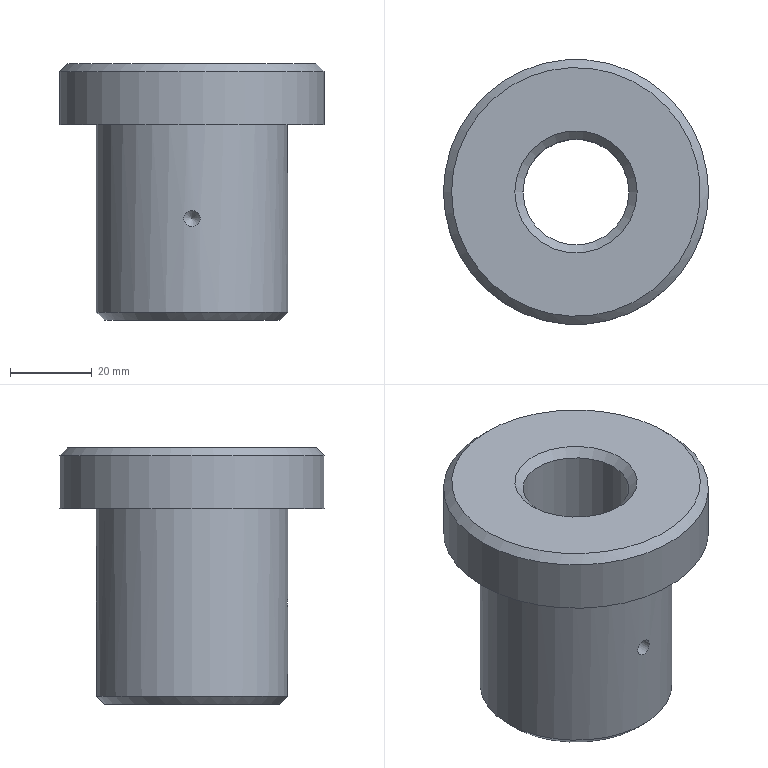Component | NX | BEARINGNUT | 1 solid | 12 faces | box 65 x 65 x 63 mm | volume 98521 mm3 | cone 5 | cylinder 4 | plane 3 | commonest cylinder face diameters 47 x1 65 x1 26 x1 4 x1
STEP:
#1=CARTESIAN_POINT('',(0.,0.,0.));
#2=DIRECTION('',(0.,0.,1.));
#3=DIRECTION('',(1.,0.,0.));
#4=AXIS2_PLACEMENT_3D('',#1,#2,#3);
#5=CARTESIAN_POINT('',(19.835,7.63,211.));
#6=VERTEX_POINT('',#5);
#7=CARTESIAN_POINT('',(4.835,7.63,211.));
#8=DIRECTION('',(0.,0.,1.));
#9=DIRECTION('',(1.,0.,0.));
#10=AXIS2_PLACEMENT_3D('',#7,#8,#9);
#11=CIRCLE('',#10,15.);
#12=CARTESIAN_POINT('',(4.835,7.63,211.));
#13=DIRECTION('',(0.,0.,-1.));
#14=DIRECTION('',(1.,0.,0.));
#15=AXIS2_PLACEMENT_3D('',#12,#13,#14);
#16=PLANE('',#15);
#17=CARTESIAN_POINT('',(15.,-0.));
#18=CARTESIAN_POINT('',(15.,-25.981));
#19=CARTESIAN_POINT('',(-7.5,-12.99));
#20=CARTESIAN_POINT('',(-30.,-0.));
#21=CARTESIAN_POINT('',(-7.5,12.99));
#22=CARTESIAN_POINT('',(15.,25.981));
#23=CARTESIAN_POINT('',(15.,-0.));
#24=(BOUNDED_CURVE()B_SPLINE_CURVE(2,(#17,#18,#19,#20,#21,#22,#23),.UNSPECIFIED.,.T.,.F.)B_SPLINE_CURVE_WITH_KNOTS((1,2,2,2,2,1),(-2.094,0.,2.094,4.189,6.283,8.378),.UNSPECIFIED.)CURVE()GEOMETRIC_REPRESENTATION_ITEM()RATIONAL_B_SPLINE_CURVE((1.,0.5,1.,0.5,1.,0.5,1.))REPRESENTATION_ITEM(''));
#25=(GEOMETRIC_REPRESENTATION_CONTEXT(2)PARAMETRIC_REPRESENTATION_CONTEXT()REPRESENTATION_CONTEXT('',''));
#26=DEFINITIONAL_REPRESENTATION('',(#24),#25);
#27=PCURVE('',#16,#26);
#28=CARTESIAN_POINT('',(4.835,7.63,213.));
#29=DIRECTION('',(0.,0.,-1.));
#30=DIRECTION('',(1.,0.,0.));
#31=AXIS2_PLACEMENT_3D('',#28,#29,#30);
#32=CONICAL_SURFACE('',#31,13.,0.7854);
#33=CARTESIAN_POINT('',(6.283,2.));
#34=DIRECTION('',(-1.,0.));
#35=VECTOR('',#34,1.);
#36=LINE('',#33,#35);
#37=(GEOMETRIC_REPRESENTATION_CONTEXT(2)PARAMETRIC_REPRESENTATION_CONTEXT()REPRESENTATION_CONTEXT('',''));
#38=DEFINITIONAL_REPRESENTATION('',(#36),#37);
#39=PCURVE('',#32,#38);
#40=SURFACE_CURVE('',#11,(#27,#39),.PCURVE_S1.);
#41=EDGE_CURVE('',#6,#6,#40,.T.);
#42=ORIENTED_EDGE('',*,*,#41,.T.);
#43=EDGE_LOOP('',(#42));
#44=FACE_BOUND('',#43,.T.);
#45=CARTESIAN_POINT('',(26.335,7.63,211.));
#46=VERTEX_POINT('',#45);
#47=CARTESIAN_POINT('',(4.835,7.63,211.));
#48=DIRECTION('',(0.,0.,-1.));
#49=DIRECTION('',(1.,0.,0.));
#50=AXIS2_PLACEMENT_3D('',#47,#48,#49);
#51=CIRCLE('',#50,21.5);
#52=CARTESIAN_POINT('',(0.,0.));
#53=DIRECTION('',(1.,0.));
#54=AXIS2_PLACEMENT_2D('',#52,#53);
#55=CIRCLE('',#54,21.5);
#56=(GEOMETRIC_REPRESENTATION_CONTEXT(2)PARAMETRIC_REPRESENTATION_CONTEXT()REPRESENTATION_CONTEXT('',''));
#57=DEFINITIONAL_REPRESENTATION('',(#55),#56);
#58=PCURVE('',#16,#57);
#59=CARTESIAN_POINT('',(4.835,7.63,213.));
#60=DIRECTION('',(0.,0.,1.));
#61=DIRECTION('',(-1.,0.,0.));
#62=AXIS2_PLACEMENT_3D('',#59,#60,#61);
#63=CONICAL_SURFACE('',#62,23.5,0.7854);
#64=CARTESIAN_POINT('',(9.425,-2.));
#65=DIRECTION('',(-1.,0.));
#66=VECTOR('',#65,1.);
#67=LINE('',#64,#66);
#68=(GEOMETRIC_REPRESENTATION_CONTEXT(2)PARAMETRIC_REPRESENTATION_CONTEXT()REPRESENTATION_CONTEXT('',''));
#69=DEFINITIONAL_REPRESENTATION('',(#67),#68);
#70=PCURVE('',#63,#69);
#71=SURFACE_CURVE('',#51,(#58,#70),.PCURVE_S1.);
#72=EDGE_CURVE('',#46,#46,#71,.T.);
#73=ORIENTED_EDGE('',*,*,#72,.T.);
#74=EDGE_LOOP('',(#73));
#75=FACE_BOUND('',#74,.T.);
#76=ADVANCED_FACE('',(#44,#75),#16,.T.);
#77=CARTESIAN_POINT('',(28.335,7.63,213.));
#78=VERTEX_POINT('',#77);
#79=CARTESIAN_POINT('',(-18.665,7.63,213.));
#80=VERTEX_POINT('',#79);
#81=CARTESIAN_POINT('',(4.835,7.63,213.));
#82=DIRECTION('',(0.,0.,1.));
#83=DIRECTION('',(1.,0.,0.));
#84=AXIS2_PLACEMENT_3D('',#81,#82,#83);
#85=CIRCLE('',#84,23.5);
#86=CARTESIAN_POINT('',(4.835,7.63,211.));
#87=DIRECTION('',(0.,0.,1.));
#88=DIRECTION('',(-1.,0.,0.));
#89=AXIS2_PLACEMENT_3D('',#86,#87,#88);
#90=CYLINDRICAL_SURFACE('',#89,23.5);
#91=CARTESIAN_POINT('',(3.142,2.));
#92=DIRECTION('',(1.,0.));
#93=VECTOR('',#92,1.);
#94=LINE('',#91,#93);
#95=(GEOMETRIC_REPRESENTATION_CONTEXT(2)PARAMETRIC_REPRESENTATION_CONTEXT()REPRESENTATION_CONTEXT('',''));
#96=DEFINITIONAL_REPRESENTATION('',(#94),#95);
#97=PCURVE('',#90,#96);
#98=CARTESIAN_POINT('',(3.142,0.));
#99=DIRECTION('',(1.,0.));
#100=VECTOR('',#99,1.);
#101=LINE('',#98,#100);
#102=(GEOMETRIC_REPRESENTATION_CONTEXT(2)PARAMETRIC_REPRESENTATION_CONTEXT()REPRESENTATION_CONTEXT('',''));
#103=DEFINITIONAL_REPRESENTATION('',(#101),#102);
#104=PCURVE('',#63,#103);
#105=SURFACE_CURVE('',#85,(#97,#104),.PCURVE_S1.);
#106=EDGE_CURVE('',#78,#80,#105,.T.);
#107=ORIENTED_EDGE('',*,*,#106,.T.);
#108=CARTESIAN_POINT('',(-18.665,7.63,259.));
#109=VERTEX_POINT('',#108);
#110=CARTESIAN_POINT('',(-18.665,7.63,213.));
#111=CARTESIAN_POINT('',(-18.665,7.63,259.));
#112=B_SPLINE_CURVE_WITH_KNOTS('',1,(#110,#111),.UNSPECIFIED.,.F.,.F.,(2,2),(2.,48.),.PIECEWISE_BEZIER_KNOTS.);
#113=CARTESIAN_POINT('',(6.283,0.));
#114=DIRECTION('',(0.,1.));
#115=VECTOR('',#114,1.);
#116=LINE('',#113,#115);
#117=(GEOMETRIC_REPRESENTATION_CONTEXT(2)PARAMETRIC_REPRESENTATION_CONTEXT()REPRESENTATION_CONTEXT('',''));
#118=DEFINITIONAL_REPRESENTATION('',(#116),#117);
#119=PCURVE('',#90,#118);
#120=CARTESIAN_POINT('',(0.,0.));
#121=DIRECTION('',(0.,1.));
#122=VECTOR('',#121,1.);
#123=LINE('',#120,#122);
#124=(GEOMETRIC_REPRESENTATION_CONTEXT(2)PARAMETRIC_REPRESENTATION_CONTEXT()REPRESENTATION_CONTEXT('',''));
#125=DEFINITIONAL_REPRESENTATION('',(#123),#124);
#126=PCURVE('',#90,#125);
#127=SEAM_CURVE('',#112,(#119,#126),.PCURVE_S1.);
#128=EDGE_CURVE('',#80,#109,#127,.T.);
#129=ORIENTED_EDGE('',*,*,#128,.T.);
#130=CARTESIAN_POINT('',(4.835,7.63,259.));
#131=DIRECTION('',(0.,0.,-1.));
#132=DIRECTION('',(-1.,0.,0.));
#133=AXIS2_PLACEMENT_3D('',#130,#131,#132);
#134=CIRCLE('',#133,23.5);
#135=CARTESIAN_POINT('',(6.283,48.));
#136=DIRECTION('',(-1.,0.));
#137=VECTOR('',#136,1.);
#138=LINE('',#135,#137);
#139=(GEOMETRIC_REPRESENTATION_CONTEXT(2)PARAMETRIC_REPRESENTATION_CONTEXT()REPRESENTATION_CONTEXT('',''));
#140=DEFINITIONAL_REPRESENTATION('',(#138),#139);
#141=PCURVE('',#90,#140);
#142=CARTESIAN_POINT('',(4.835,7.63,259.));
#143=DIRECTION('',(0.,0.,-1.));
#144=DIRECTION('',(1.,0.,0.));
#145=AXIS2_PLACEMENT_3D('',#142,#143,#144);
#146=PLANE('',#145);
#147=CARTESIAN_POINT('',(0.,0.));
#148=DIRECTION('',(-1.,0.));
#149=AXIS2_PLACEMENT_2D('',#147,#148);
#150=CIRCLE('',#149,23.5);
#151=(GEOMETRIC_REPRESENTATION_CONTEXT(2)PARAMETRIC_REPRESENTATION_CONTEXT()REPRESENTATION_CONTEXT('',''));
#152=DEFINITIONAL_REPRESENTATION('',(#150),#151);
#153=PCURVE('',#146,#152);
#154=SURFACE_CURVE('',#134,(#141,#153),.PCURVE_S1.);
#155=EDGE_CURVE('',#109,#109,#154,.T.);
#156=ORIENTED_EDGE('',*,*,#155,.T.);
#157=ORIENTED_EDGE('',*,*,#128,.F.);
#158=CARTESIAN_POINT('',(4.835,7.63,213.));
#159=DIRECTION('',(0.,0.,1.));
#160=DIRECTION('',(1.,0.,0.));
#161=AXIS2_PLACEMENT_3D('',#158,#159,#160);
#162=CIRCLE('',#161,23.5);
#163=CARTESIAN_POINT('',(-3.142,2.));
#164=DIRECTION('',(1.,0.));
#165=VECTOR('',#164,1.);
#166=LINE('',#163,#165);
#167=(GEOMETRIC_REPRESENTATION_CONTEXT(2)PARAMETRIC_REPRESENTATION_CONTEXT()REPRESENTATION_CONTEXT('',''));
#168=DEFINITIONAL_REPRESENTATION('',(#166),#167);
#169=PCURVE('',#90,#168);
#170=CARTESIAN_POINT('',(3.142,0.));
#171=DIRECTION('',(1.,0.));
#172=VECTOR('',#171,1.);
#173=LINE('',#170,#172);
#174=(GEOMETRIC_REPRESENTATION_CONTEXT(2)PARAMETRIC_REPRESENTATION_CONTEXT()REPRESENTATION_CONTEXT('',''));
#175=DEFINITIONAL_REPRESENTATION('',(#173),#174);
#176=PCURVE('',#63,#175);
#177=SURFACE_CURVE('',#162,(#169,#176),.PCURVE_S1.);
#178=EDGE_CURVE('',#80,#78,#177,.T.);
#179=ORIENTED_EDGE('',*,*,#178,.T.);
#180=EDGE_LOOP('',(#107,#129,#156,#157,#179));
#181=FACE_BOUND('',#180,.T.);
#182=CARTESIAN_POINT('',(4.835,-15.87,234.));
#183=VERTEX_POINT('',#182);
#184=CARTESIAN_POINT('',(4.835,-15.87,234.));
#185=CARTESIAN_POINT('',(5.059,-15.87,234.));
#186=CARTESIAN_POINT('',(5.285,-15.866,234.038));
#187=CARTESIAN_POINT('',(5.496,-15.86,234.112));
#188=CARTESIAN_POINT('',(5.707,-15.854,234.186));
#189=CARTESIAN_POINT('',(5.908,-15.846,234.297));
#190=CARTESIAN_POINT('',(6.082,-15.837,234.436));
#191=CARTESIAN_POINT('',(6.257,-15.827,234.576));
#192=CARTESIAN_POINT('',(6.41,-15.817,234.747));
#193=CARTESIAN_POINT('',(6.529,-15.808,234.937));
#194=CARTESIAN_POINT('',(6.648,-15.8,235.126));
#195=CARTESIAN_POINT('',(6.736,-15.793,235.339));
#196=CARTESIAN_POINT('',(6.786,-15.789,235.558));
#197=CARTESIAN_POINT('',(6.835,-15.784,235.776));
#198=CARTESIAN_POINT('',(6.848,-15.783,236.006));
#199=CARTESIAN_POINT('',(6.822,-15.785,236.228));
#200=CARTESIAN_POINT('',(6.797,-15.788,236.45));
#201=CARTESIAN_POINT('',(6.733,-15.793,236.67));
#202=CARTESIAN_POINT('',(6.636,-15.801,236.871));
#203=CARTESIAN_POINT('',(6.539,-15.808,237.072));
#204=CARTESIAN_POINT('',(6.405,-15.818,237.259));
#205=CARTESIAN_POINT('',(6.247,-15.827,237.416));
#206=CARTESIAN_POINT('',(6.089,-15.837,237.574));
#207=CARTESIAN_POINT('',(5.901,-15.846,237.707));
#208=CARTESIAN_POINT('',(5.699,-15.854,237.804));
#209=CARTESIAN_POINT('',(5.497,-15.861,237.901));
#210=CARTESIAN_POINT('',(5.275,-15.867,237.964));
#211=CARTESIAN_POINT('',(5.052,-15.869,237.988));
#212=CARTESIAN_POINT('',(4.83,-15.871,238.012));
#213=CARTESIAN_POINT('',(4.601,-15.869,237.999));
#214=CARTESIAN_POINT('',(4.383,-15.865,237.948));
#215=CARTESIAN_POINT('',(4.166,-15.861,237.898));
#216=CARTESIAN_POINT('',(3.955,-15.854,237.809));
#217=CARTESIAN_POINT('',(3.766,-15.845,237.69));
#218=CARTESIAN_POINT('',(3.577,-15.837,237.571));
#219=CARTESIAN_POINT('',(3.406,-15.827,237.417));
#220=CARTESIAN_POINT('',(3.268,-15.817,237.242));
#221=CARTESIAN_POINT('',(3.129,-15.808,237.067));
#222=CARTESIAN_POINT('',(3.018,-15.799,236.864));
#223=CARTESIAN_POINT('',(2.945,-15.793,236.653));
#224=CARTESIAN_POINT('',(2.872,-15.788,236.441));
#225=CARTESIAN_POINT('',(2.834,-15.784,236.214));
#226=CARTESIAN_POINT('',(2.835,-15.784,235.99));
#227=CARTESIAN_POINT('',(2.836,-15.784,235.767));
#228=CARTESIAN_POINT('',(2.876,-15.788,235.541));
#229=CARTESIAN_POINT('',(2.951,-15.794,235.33));
#230=CARTESIAN_POINT('',(3.025,-15.8,235.12));
#231=CARTESIAN_POINT('',(3.137,-15.809,234.92));
#232=CARTESIAN_POINT('',(3.277,-15.818,234.746));
#233=CARTESIAN_POINT('',(3.417,-15.827,234.572));
#234=CARTESIAN_POINT('',(3.589,-15.837,234.419));
#235=CARTESIAN_POINT('',(3.779,-15.846,234.301));
#236=CARTESIAN_POINT('',(3.97,-15.854,234.183));
#237=CARTESIAN_POINT('',(4.183,-15.862,234.096));
#238=CARTESIAN_POINT('',(4.402,-15.866,234.047));
#239=CARTESIAN_POINT('',(4.544,-15.868,234.016));
#240=CARTESIAN_POINT('',(4.69,-15.87,234.));
#241=CARTESIAN_POINT('',(4.835,-15.87,234.));
#242=B_SPLINE_CURVE_WITH_KNOTS('',3,(#184,#185,#186,#187,#188,#189,#190,#191,#192,#193,#194,#195,#196,#197,#198,#199,#200,#201,#202,#203,#204,#205,#206,#207,#208,#209,#210,#211,#212,#213,#214,#215,#216,#217,#218,#219,#220,#221,#222,#223,#224,#225,#226,#227,#228,#229,#230,#231,#232,#233,#234,#235,#236,#237,#238,#239,#240,#241),.UNSPECIFIED.,.T.,.F.,(1,3,3,3,3,3,3,3,3,3,3,3,3,3,3,3,3,3,3,3,3,1),(-0.03454,0.,0.05357,0.1071,0.1608,0.2146,0.2682,0.3217,0.3753,0.429,0.4828,0.5364,0.5899,0.6435,0.6973,0.751,0.8045,0.858,0.9117,0.9655,1.,1.054),.UNSPECIFIED.);
#243=CARTESIAN_POINT('',(1.571,23.));
#244=CARTESIAN_POINT('',(1.573,23.));
#245=CARTESIAN_POINT('',(1.577,23.003));
#246=CARTESIAN_POINT('',(1.583,23.019));
#247=CARTESIAN_POINT('',(1.589,23.044));
#248=CARTESIAN_POINT('',(1.595,23.08));
#249=CARTESIAN_POINT('',(1.601,23.124));
#250=CARTESIAN_POINT('',(1.606,23.179));
#251=CARTESIAN_POINT('',(1.612,23.243));
#252=CARTESIAN_POINT('',(1.617,23.316));
#253=CARTESIAN_POINT('',(1.622,23.398));
#254=CARTESIAN_POINT('',(1.627,23.487));
#255=CARTESIAN_POINT('',(1.631,23.584));
#256=CARTESIAN_POINT('',(1.635,23.689));
#257=CARTESIAN_POINT('',(1.639,23.8));
#258=CARTESIAN_POINT('',(1.643,23.917));
#259=CARTESIAN_POINT('',(1.646,24.04));
#260=CARTESIAN_POINT('',(1.648,24.168));
#261=CARTESIAN_POINT('',(1.651,24.3));
#262=CARTESIAN_POINT('',(1.653,24.436));
#263=CARTESIAN_POINT('',(1.654,24.574));
#264=CARTESIAN_POINT('',(1.655,24.714));
#265=CARTESIAN_POINT('',(1.656,24.856));
#266=CARTESIAN_POINT('',(1.656,25.));
#267=CARTESIAN_POINT('',(1.656,25.143));
#268=CARTESIAN_POINT('',(1.655,25.284));
#269=CARTESIAN_POINT('',(1.654,25.425));
#270=CARTESIAN_POINT('',(1.653,25.563));
#271=CARTESIAN_POINT('',(1.651,25.699));
#272=CARTESIAN_POINT('',(1.648,25.831));
#273=CARTESIAN_POINT('',(1.646,25.958));
#274=CARTESIAN_POINT('',(1.643,26.081));
#275=CARTESIAN_POINT('',(1.639,26.199));
#276=CARTESIAN_POINT('',(1.635,26.31));
#277=CARTESIAN_POINT('',(1.631,26.415));
#278=CARTESIAN_POINT('',(1.627,26.512));
#279=CARTESIAN_POINT('',(1.622,26.602));
#280=CARTESIAN_POINT('',(1.617,26.683));
#281=CARTESIAN_POINT('',(1.612,26.756));
#282=CARTESIAN_POINT('',(1.606,26.82));
#283=CARTESIAN_POINT('',(1.601,26.875));
#284=CARTESIAN_POINT('',(1.595,26.92));
#285=CARTESIAN_POINT('',(1.589,26.956));
#286=CARTESIAN_POINT('',(1.583,26.981));
#287=CARTESIAN_POINT('',(1.577,26.996));
#288=CARTESIAN_POINT('',(1.571,27.002));
#289=CARTESIAN_POINT('',(1.565,26.996));
#290=CARTESIAN_POINT('',(1.559,26.981));
#291=CARTESIAN_POINT('',(1.553,26.956));
#292=CARTESIAN_POINT('',(1.547,26.921));
#293=CARTESIAN_POINT('',(1.541,26.876));
#294=CARTESIAN_POINT('',(1.535,26.821));
#295=CARTESIAN_POINT('',(1.53,26.757));
#296=CARTESIAN_POINT('',(1.525,26.685));
#297=CARTESIAN_POINT('',(1.52,26.603));
#298=CARTESIAN_POINT('',(1.515,26.514));
#299=CARTESIAN_POINT('',(1.511,26.416));
#300=CARTESIAN_POINT('',(1.506,26.312));
#301=CARTESIAN_POINT('',(1.503,26.201));
#302=CARTESIAN_POINT('',(1.499,26.084));
#303=CARTESIAN_POINT('',(1.496,25.961));
#304=CARTESIAN_POINT('',(1.493,25.833));
#305=CARTESIAN_POINT('',(1.491,25.701));
#306=CARTESIAN_POINT('',(1.489,25.566));
#307=CARTESIAN_POINT('',(1.487,25.428));
#308=CARTESIAN_POINT('',(1.486,25.287));
#309=CARTESIAN_POINT('',(1.486,25.144));
#310=CARTESIAN_POINT('',(1.486,25.002));
#311=CARTESIAN_POINT('',(1.486,24.859));
#312=CARTESIAN_POINT('',(1.486,24.717));
#313=CARTESIAN_POINT('',(1.487,24.576));
#314=CARTESIAN_POINT('',(1.489,24.437));
#315=CARTESIAN_POINT('',(1.491,24.302));
#316=CARTESIAN_POINT('',(1.493,24.17));
#317=CARTESIAN_POINT('',(1.496,24.042));
#318=CARTESIAN_POINT('',(1.499,23.919));
#319=CARTESIAN_POINT('',(1.503,23.802));
#320=CARTESIAN_POINT('',(1.506,23.691));
#321=CARTESIAN_POINT('',(1.51,23.586));
#322=CARTESIAN_POINT('',(1.515,23.489));
#323=CARTESIAN_POINT('',(1.52,23.399));
#324=CARTESIAN_POINT('',(1.525,23.317));
#325=CARTESIAN_POINT('',(1.53,23.245));
#326=CARTESIAN_POINT('',(1.535,23.18));
#327=CARTESIAN_POINT('',(1.541,23.126));
#328=CARTESIAN_POINT('',(1.547,23.08));
#329=CARTESIAN_POINT('',(1.553,23.045));
#330=CARTESIAN_POINT('',(1.559,23.019));
#331=CARTESIAN_POINT('',(1.565,23.003));
#332=CARTESIAN_POINT('',(1.569,23.));
#333=CARTESIAN_POINT('',(1.571,23.));
#334=B_SPLINE_CURVE_WITH_KNOTS('',3,(#243,#244,#245,#246,#247,#248,#249,#250,#251,#252,#253,#254,#255,#256,#257,#258,#259,#260,#261,#262,#263,#264,#265,#266,#267,#268,#269,#270,#271,#272,#273,#274,#275,#276,#277,#278,#279,#280,#281,#282,#283,#284,#285,#286,#287,#288,#289,#290,#291,#292,#293,#294,#295,#296,#297,#298,#299,#300,#301,#302,#303,#304,#305,#306,#307,#308,#309,#310,#311,#312,#313,#314,#315,#316,#317,#318,#319,#320,#321,#322,#323,#324,#325,#326,#327,#328,#329,#330,#331,#332,#333),.UNSPECIFIED.,.T.,.F.,(4,1,1,1,1,1,1,1,1,1,1,1,1,1,1,1,1,1,1,1,1,1,1,1,1,1,1,1,1,1,1,1,1,1,1,1,1,1,1,1,1,1,1,1,1,1,1,1,1,1,1,1,1,1,1,1,1,1,1,1,1,1,1,1,1,1,1,1,1,1,1,1,1,1,1,1,1,1,1,1,1,1,1,1,1,1,1,1,4),(0.,0.01136,0.02273,0.03409,0.04545,0.05682,0.06818,0.07955,0.09091,0.1023,0.1136,0.125,0.1364,0.1477,0.1591,0.1705,0.1818,0.1932,0.2045,0.2159,0.2273,0.2386,0.25,0.2614,0.2727,0.2841,0.2955,0.3068,0.3182,0.3295,0.3409,0.3523,0.3636,0.375,0.3864,0.3977,0.4091,0.4205,0.4318,0.4432,0.4545,0.4659,0.4773,0.4886,0.5,0.5114,0.5227,0.5341,0.5455,0.5568,0.5682,0.5795,0.5909,0.6023,0.6136,0.625,0.6364,0.6477,0.6591,0.6705,0.6818,0.6932,0.7045,0.7159,0.7273,0.7386,0.75,0.7614,0.7727,0.7841,0.7955,0.8068,0.8182,0.8295,0.8409,0.8523,0.8636,0.875,0.8864,0.8977,0.9091,0.9205,0.9318,0.9432,0.9545,0.9659,0.9773,0.9886,1.),.QUASI_UNIFORM_KNOTS.);
#335=(GEOMETRIC_REPRESENTATION_CONTEXT(2)PARAMETRIC_REPRESENTATION_CONTEXT()REPRESENTATION_CONTEXT('',''));
#336=DEFINITIONAL_REPRESENTATION('',(#334),#335);
#337=PCURVE('',#90,#336);
#338=CARTESIAN_POINT('',(4.835,-70.37,236.));
#339=DIRECTION('',(0.,1.,0.));
#340=DIRECTION('',(0.,0.,-1.));
#341=AXIS2_PLACEMENT_3D('',#338,#339,#340);
#342=CYLINDRICAL_SURFACE('',#341,2.);
#343=CARTESIAN_POINT('',(6.283,54.5));
#344=CARTESIAN_POINT('',(6.259,54.5));
#345=CARTESIAN_POINT('',(6.212,54.5));
#346=CARTESIAN_POINT('',(6.14,54.502));
#347=CARTESIAN_POINT('',(6.069,54.504));
#348=CARTESIAN_POINT('',(5.997,54.507));
#349=CARTESIAN_POINT('',(5.926,54.51));
#350=CARTESIAN_POINT('',(5.855,54.515));
#351=CARTESIAN_POINT('',(5.783,54.519));
#352=CARTESIAN_POINT('',(5.712,54.525));
#353=CARTESIAN_POINT('',(5.64,54.531));
#354=CARTESIAN_POINT('',(5.569,54.536));
#355=CARTESIAN_POINT('',(5.498,54.543));
#356=CARTESIAN_POINT('',(5.427,54.549));
#357=CARTESIAN_POINT('',(5.355,54.555));
#358=CARTESIAN_POINT('',(5.284,54.56));
#359=CARTESIAN_POINT('',(5.213,54.566));
#360=CARTESIAN_POINT('',(5.141,54.571));
#361=CARTESIAN_POINT('',(5.07,54.575));
#362=CARTESIAN_POINT('',(4.998,54.579));
#363=CARTESIAN_POINT('',(4.927,54.582));
#364=CARTESIAN_POINT('',(4.856,54.584));
#365=CARTESIAN_POINT('',(4.784,54.585));
#366=CARTESIAN_POINT('',(4.713,54.585));
#367=CARTESIAN_POINT('',(4.641,54.585));
#368=CARTESIAN_POINT('',(4.57,54.584));
#369=CARTESIAN_POINT('',(4.499,54.582));
#370=CARTESIAN_POINT('',(4.427,54.579));
#371=CARTESIAN_POINT('',(4.355,54.575));
#372=CARTESIAN_POINT('',(4.284,54.571));
#373=CARTESIAN_POINT('',(4.213,54.566));
#374=CARTESIAN_POINT('',(4.142,54.56));
#375=CARTESIAN_POINT('',(4.07,54.555));
#376=CARTESIAN_POINT('',(3.999,54.549));
#377=CARTESIAN_POINT('',(3.927,54.543));
#378=CARTESIAN_POINT('',(3.856,54.537));
#379=CARTESIAN_POINT('',(3.785,54.531));
#380=CARTESIAN_POINT('',(3.713,54.525));
#381=CARTESIAN_POINT('',(3.642,54.52));
#382=CARTESIAN_POINT('',(3.571,54.515));
#383=CARTESIAN_POINT('',(3.499,54.51));
#384=CARTESIAN_POINT('',(3.428,54.507));
#385=CARTESIAN_POINT('',(3.356,54.504));
#386=CARTESIAN_POINT('',(3.285,54.502));
#387=CARTESIAN_POINT('',(3.214,54.5));
#388=CARTESIAN_POINT('',(3.142,54.5));
#389=CARTESIAN_POINT('',(3.071,54.5));
#390=CARTESIAN_POINT('',(2.999,54.502));
#391=CARTESIAN_POINT('',(2.928,54.504));
#392=CARTESIAN_POINT('',(2.857,54.507));
#393=CARTESIAN_POINT('',(2.785,54.51));
#394=CARTESIAN_POINT('',(2.714,54.515));
#395=CARTESIAN_POINT('',(2.642,54.519));
#396=CARTESIAN_POINT('',(2.571,54.525));
#397=CARTESIAN_POINT('',(2.5,54.53));
#398=CARTESIAN_POINT('',(2.428,54.536));
#399=CARTESIAN_POINT('',(2.357,54.543));
#400=CARTESIAN_POINT('',(2.285,54.549));
#401=CARTESIAN_POINT('',(2.214,54.555));
#402=CARTESIAN_POINT('',(2.143,54.56));
#403=CARTESIAN_POINT('',(2.071,54.566));
#404=CARTESIAN_POINT('',(2.,54.571));
#405=CARTESIAN_POINT('',(1.929,54.575));
#406=CARTESIAN_POINT('',(1.858,54.579));
#407=CARTESIAN_POINT('',(1.786,54.581));
#408=CARTESIAN_POINT('',(1.714,54.584));
#409=CARTESIAN_POINT('',(1.643,54.585));
#410=CARTESIAN_POINT('',(1.572,54.585));
#411=CARTESIAN_POINT('',(1.501,54.585));
#412=CARTESIAN_POINT('',(1.429,54.584));
#413=CARTESIAN_POINT('',(1.357,54.582));
#414=CARTESIAN_POINT('',(1.286,54.579));
#415=CARTESIAN_POINT('',(1.215,54.575));
#416=CARTESIAN_POINT('',(1.143,54.571));
#417=CARTESIAN_POINT('',(1.072,54.566));
#418=CARTESIAN_POINT('',(1.,54.56));
#419=CARTESIAN_POINT('',(0.929,54.555));
#420=CARTESIAN_POINT('',(0.858,54.549));
#421=CARTESIAN_POINT('',(0.7866,54.543));
#422=CARTESIAN_POINT('',(0.7151,54.537));
#423=CARTESIAN_POINT('',(0.6435,54.531));
#424=CARTESIAN_POINT('',(0.5723,54.525));
#425=CARTESIAN_POINT('',(0.5012,54.52));
#426=CARTESIAN_POINT('',(0.4297,54.515));
#427=CARTESIAN_POINT('',(0.3582,54.51));
#428=CARTESIAN_POINT('',(0.2866,54.507));
#429=CARTESIAN_POINT('',(0.2156,54.504));
#430=CARTESIAN_POINT('',(0.1436,54.502));
#431=CARTESIAN_POINT('',(0.07178,54.5));
#432=CARTESIAN_POINT('',(0.02389,54.5));
#433=CARTESIAN_POINT('',(0.,54.5));
#434=B_SPLINE_CURVE_WITH_KNOTS('',3,(#343,#344,#345,#346,#347,#348,#349,#350,#351,#352,#353,#354,#355,#356,#357,#358,#359,#360,#361,#362,#363,#364,#365,#366,#367,#368,#369,#370,#371,#372,#373,#374,#375,#376,#377,#378,#379,#380,#381,#382,#383,#384,#385,#386,#387,#388,#389,#390,#391,#392,#393,#394,#395,#396,#397,#398,#399,#400,#401,#402,#403,#404,#405,#406,#407,#408,#409,#410,#411,#412,#413,#414,#415,#416,#417,#418,#419,#420,#421,#422,#423,#424,#425,#426,#427,#428,#429,#430,#431,#432,#433),.UNSPECIFIED.,.F.,.F.,(4,1,1,1,1,1,1,1,1,1,1,1,1,1,1,1,1,1,1,1,1,1,1,1,1,1,1,1,1,1,1,1,1,1,1,1,1,1,1,1,1,1,1,1,1,1,1,1,1,1,1,1,1,1,1,1,1,1,1,1,1,1,1,1,1,1,1,1,1,1,1,1,1,1,1,1,1,1,1,1,1,1,1,1,1,1,1,1,4),(0.,0.01136,0.02273,0.03409,0.04545,0.05682,0.06818,0.07955,0.09091,0.1023,0.1136,0.125,0.1364,0.1477,0.1591,0.1705,0.1818,0.1932,0.2045,0.2159,0.2273,0.2386,0.25,0.2614,0.2727,0.2841,0.2955,0.3068,0.3182,0.3295,0.3409,0.3523,0.3636,0.375,0.3864,0.3977,0.4091,0.4205,0.4318,0.4432,0.4545,0.4659,0.4773,0.4886,0.5,0.5114,0.5227,0.5341,0.5455,0.5568,0.5682,0.5795,0.5909,0.6023,0.6136,0.625,0.6364,0.6477,0.6591,0.6705,0.6818,0.6932,0.7045,0.7159,0.7273,0.7386,0.75,0.7614,0.7727,0.7841,0.7955,0.8068,0.8182,0.8295,0.8409,0.8523,0.8636,0.875,0.8864,0.8977,0.9091,0.9205,0.9318,0.9432,0.9545,0.9659,0.9773,0.9886,1.),.QUASI_UNIFORM_KNOTS.);
#435=(GEOMETRIC_REPRESENTATION_CONTEXT(2)PARAMETRIC_REPRESENTATION_CONTEXT()REPRESENTATION_CONTEXT('',''));
#436=DEFINITIONAL_REPRESENTATION('',(#434),#435);
#437=PCURVE('',#342,#436);
#438=SURFACE_CURVE('',#242,(#337,#437),.PCURVE_S1.);
#439=EDGE_CURVE('',#183,#183,#438,.T.);
#440=ORIENTED_EDGE('',*,*,#439,.F.);
#441=EDGE_LOOP('',(#440));
#442=FACE_BOUND('',#441,.T.);
#443=ADVANCED_FACE('',(#181,#442),#90,.T.);
#444=CARTESIAN_POINT('',(-10.165,7.63,274.));
#445=VERTEX_POINT('',#444);
#446=CARTESIAN_POINT('',(4.835,7.63,274.));
#447=DIRECTION('',(0.,0.,-1.));
#448=DIRECTION('',(-1.,0.,0.));
#449=AXIS2_PLACEMENT_3D('',#446,#447,#448);
#450=CIRCLE('',#449,15.);
#451=CARTESIAN_POINT('',(4.835,7.63,274.));
#452=DIRECTION('',(0.,0.,1.));
#453=DIRECTION('',(-1.,0.,0.));
#454=AXIS2_PLACEMENT_3D('',#451,#452,#453);
#455=PLANE('',#454);
#456=CARTESIAN_POINT('',(15.,-0.));
#457=CARTESIAN_POINT('',(15.,-25.981));
#458=CARTESIAN_POINT('',(-7.5,-12.99));
#459=CARTESIAN_POINT('',(-30.,-0.));
#460=CARTESIAN_POINT('',(-7.5,12.99));
#461=CARTESIAN_POINT('',(15.,25.981));
#462=CARTESIAN_POINT('',(15.,-0.));
#463=(BOUNDED_CURVE()B_SPLINE_CURVE(2,(#456,#457,#458,#459,#460,#461,#462),.UNSPECIFIED.,.T.,.F.)B_SPLINE_CURVE_WITH_KNOTS((1,2,2,2,2,1),(-2.094,0.,2.094,4.189,6.283,8.378),.UNSPECIFIED.)CURVE()GEOMETRIC_REPRESENTATION_ITEM()RATIONAL_B_SPLINE_CURVE((1.,0.5,1.,0.5,1.,0.5,1.))REPRESENTATION_ITEM(''));
#464=(GEOMETRIC_REPRESENTATION_CONTEXT(2)PARAMETRIC_REPRESENTATION_CONTEXT()REPRESENTATION_CONTEXT('',''));
#465=DEFINITIONAL_REPRESENTATION('',(#463),#464);
#466=PCURVE('',#455,#465);
#467=CARTESIAN_POINT('',(4.835,7.63,272.));
#468=DIRECTION('',(0.,0.,1.));
#469=DIRECTION('',(-1.,0.,0.));
#470=AXIS2_PLACEMENT_3D('',#467,#468,#469);
#471=CONICAL_SURFACE('',#470,13.,0.7854);
#472=CARTESIAN_POINT('',(6.283,2.));
#473=DIRECTION('',(-1.,0.));
#474=VECTOR('',#473,1.);
#475=LINE('',#472,#474);
#476=(GEOMETRIC_REPRESENTATION_CONTEXT(2)PARAMETRIC_REPRESENTATION_CONTEXT()REPRESENTATION_CONTEXT('',''));
#477=DEFINITIONAL_REPRESENTATION('',(#475),#476);
#478=PCURVE('',#471,#477);
#479=SURFACE_CURVE('',#450,(#466,#478),.PCURVE_S1.);
#480=EDGE_CURVE('',#445,#445,#479,.T.);
#481=ORIENTED_EDGE('',*,*,#480,.T.);
#482=EDGE_LOOP('',(#481));
#483=FACE_BOUND('',#482,.T.);
#484=CARTESIAN_POINT('',(-25.665,7.63,274.));
#485=VERTEX_POINT('',#484);
#486=CARTESIAN_POINT('',(4.835,7.63,274.));
#487=DIRECTION('',(0.,0.,1.));
#488=DIRECTION('',(-1.,0.,0.));
#489=AXIS2_PLACEMENT_3D('',#486,#487,#488);
#490=CIRCLE('',#489,30.5);
#491=CARTESIAN_POINT('',(0.,0.));
#492=DIRECTION('',(1.,0.));
#493=AXIS2_PLACEMENT_2D('',#491,#492);
#494=CIRCLE('',#493,30.5);
#495=(GEOMETRIC_REPRESENTATION_CONTEXT(2)PARAMETRIC_REPRESENTATION_CONTEXT()REPRESENTATION_CONTEXT('',''));
#496=DEFINITIONAL_REPRESENTATION('',(#494),#495);
#497=PCURVE('',#455,#496);
#498=CARTESIAN_POINT('',(4.835,7.63,274.));
#499=DIRECTION('',(0.,0.,-1.));
#500=DIRECTION('',(1.,0.,0.));
#501=AXIS2_PLACEMENT_3D('',#498,#499,#500);
#502=CONICAL_SURFACE('',#501,30.5,0.7854);
#503=CARTESIAN_POINT('',(9.425,0.));
#504=DIRECTION('',(-1.,0.));
#505=VECTOR('',#504,1.);
#506=LINE('',#503,#505);
#507=(GEOMETRIC_REPRESENTATION_CONTEXT(2)PARAMETRIC_REPRESENTATION_CONTEXT()REPRESENTATION_CONTEXT('',''));
#508=DEFINITIONAL_REPRESENTATION('',(#506),#507);
#509=PCURVE('',#502,#508);
#510=SURFACE_CURVE('',#490,(#497,#509),.PCURVE_S1.);
#511=EDGE_CURVE('',#485,#485,#510,.T.);
#512=ORIENTED_EDGE('',*,*,#511,.T.);
#513=EDGE_LOOP('',(#512));
#514=FACE_BOUND('',#513,.T.);
#515=ADVANCED_FACE('',(#483,#514),#455,.T.);
#516=ORIENTED_EDGE('',*,*,#155,.F.);
#517=EDGE_LOOP('',(#516));
#518=FACE_BOUND('',#517,.T.);
#519=CARTESIAN_POINT('',(-27.665,7.63,259.));
#520=VERTEX_POINT('',#519);
#521=CARTESIAN_POINT('',(4.835,7.63,259.));
#522=DIRECTION('',(0.,0.,1.));
#523=DIRECTION('',(-1.,0.,0.));
#524=AXIS2_PLACEMENT_3D('',#521,#522,#523);
#525=CIRCLE('',#524,32.5);
#526=CARTESIAN_POINT('',(-32.5,0.));
#527=CARTESIAN_POINT('',(-32.5,56.292));
#528=CARTESIAN_POINT('',(16.25,28.146));
#529=CARTESIAN_POINT('',(65.,0.));
#530=CARTESIAN_POINT('',(16.25,-28.146));
#531=CARTESIAN_POINT('',(-32.5,-56.292));
#532=CARTESIAN_POINT('',(-32.5,0.));
#533=(BOUNDED_CURVE()B_SPLINE_CURVE(2,(#526,#527,#528,#529,#530,#531,#532),.UNSPECIFIED.,.T.,.F.)B_SPLINE_CURVE_WITH_KNOTS((1,2,2,2,2,1),(-2.094,0.,2.094,4.189,6.283,8.378),.UNSPECIFIED.)CURVE()GEOMETRIC_REPRESENTATION_ITEM()RATIONAL_B_SPLINE_CURVE((1.,0.5,1.,0.5,1.,0.5,1.))REPRESENTATION_ITEM(''));
#534=(GEOMETRIC_REPRESENTATION_CONTEXT(2)PARAMETRIC_REPRESENTATION_CONTEXT()REPRESENTATION_CONTEXT('',''));
#535=DEFINITIONAL_REPRESENTATION('',(#533),#534);
#536=PCURVE('',#146,#535);
#537=CARTESIAN_POINT('',(4.835,7.63,259.));
#538=DIRECTION('',(0.,0.,1.));
#539=DIRECTION('',(-1.,0.,0.));
#540=AXIS2_PLACEMENT_3D('',#537,#538,#539);
#541=CYLINDRICAL_SURFACE('',#540,32.5);
#542=CARTESIAN_POINT('',(0.,0.));
#543=DIRECTION('',(1.,0.));
#544=VECTOR('',#543,1.);
#545=LINE('',#542,#544);
#546=(GEOMETRIC_REPRESENTATION_CONTEXT(2)PARAMETRIC_REPRESENTATION_CONTEXT()REPRESENTATION_CONTEXT('',''));
#547=DEFINITIONAL_REPRESENTATION('',(#545),#546);
#548=PCURVE('',#541,#547);
#549=SURFACE_CURVE('',#525,(#536,#548),.PCURVE_S1.);
#550=EDGE_CURVE('',#520,#520,#549,.T.);
#551=ORIENTED_EDGE('',*,*,#550,.F.);
#552=EDGE_LOOP('',(#551));
#553=FACE_BOUND('',#552,.T.);
#554=ADVANCED_FACE('',(#518,#553),#146,.T.);
#555=CARTESIAN_POINT('',(-27.665,7.63,272.));
#556=VERTEX_POINT('',#555);
#557=CARTESIAN_POINT('',(4.835,7.63,272.));
#558=DIRECTION('',(0.,0.,-1.));
#559=DIRECTION('',(-1.,0.,0.));
#560=AXIS2_PLACEMENT_3D('',#557,#558,#559);
#561=CIRCLE('',#560,32.5);
#562=CARTESIAN_POINT('',(6.283,13.));
#563=DIRECTION('',(-1.,0.));
#564=VECTOR('',#563,1.);
#565=LINE('',#562,#564);
#566=(GEOMETRIC_REPRESENTATION_CONTEXT(2)PARAMETRIC_REPRESENTATION_CONTEXT()REPRESENTATION_CONTEXT('',''));
#567=DEFINITIONAL_REPRESENTATION('',(#565),#566);
#568=PCURVE('',#541,#567);
#569=CARTESIAN_POINT('',(3.142,2.));
#570=DIRECTION('',(1.,0.));
#571=VECTOR('',#570,1.);
#572=LINE('',#569,#571);
#573=(GEOMETRIC_REPRESENTATION_CONTEXT(2)PARAMETRIC_REPRESENTATION_CONTEXT()REPRESENTATION_CONTEXT('',''));
#574=DEFINITIONAL_REPRESENTATION('',(#572),#573);
#575=PCURVE('',#502,#574);
#576=SURFACE_CURVE('',#561,(#568,#575),.PCURVE_S1.);
#577=EDGE_CURVE('',#556,#556,#576,.T.);
#578=ORIENTED_EDGE('',*,*,#577,.T.);
#579=CARTESIAN_POINT('',(-27.665,7.63,259.));
#580=CARTESIAN_POINT('',(-27.665,7.63,272.));
#581=B_SPLINE_CURVE_WITH_KNOTS('',1,(#579,#580),.UNSPECIFIED.,.F.,.F.,(2,2),(0.,13.),.PIECEWISE_BEZIER_KNOTS.);
#582=CARTESIAN_POINT('',(0.,0.));
#583=DIRECTION('',(0.,1.));
#584=VECTOR('',#583,1.);
#585=LINE('',#582,#584);
#586=(GEOMETRIC_REPRESENTATION_CONTEXT(2)PARAMETRIC_REPRESENTATION_CONTEXT()REPRESENTATION_CONTEXT('',''));
#587=DEFINITIONAL_REPRESENTATION('',(#585),#586);
#588=PCURVE('',#541,#587);
#589=CARTESIAN_POINT('',(6.283,0.));
#590=DIRECTION('',(0.,1.));
#591=VECTOR('',#590,1.);
#592=LINE('',#589,#591);
#593=(GEOMETRIC_REPRESENTATION_CONTEXT(2)PARAMETRIC_REPRESENTATION_CONTEXT()REPRESENTATION_CONTEXT('',''));
#594=DEFINITIONAL_REPRESENTATION('',(#592),#593);
#595=PCURVE('',#541,#594);
#596=SEAM_CURVE('',#581,(#588,#595),.PCURVE_S1.);
#597=EDGE_CURVE('',#520,#556,#596,.T.);
#598=ORIENTED_EDGE('',*,*,#597,.F.);
#599=ORIENTED_EDGE('',*,*,#550,.T.);
#600=ORIENTED_EDGE('',*,*,#597,.T.);
#601=EDGE_LOOP('',(#578,#598,#599,#600));
#602=FACE_BOUND('',#601,.T.);
#603=ADVANCED_FACE('',(#602),#541,.T.);
#604=ORIENTED_EDGE('',*,*,#72,.F.);
#605=CARTESIAN_POINT('',(26.335,7.63,211.));
#606=CARTESIAN_POINT('',(28.335,7.63,213.));
#607=B_SPLINE_CURVE_WITH_KNOTS('',1,(#605,#606),.UNSPECIFIED.,.F.,.F.,(2,2),(-2.828,0.),.PIECEWISE_BEZIER_KNOTS.);
#608=CARTESIAN_POINT('',(9.425,0.));
#609=DIRECTION('',(0.,1.));
#610=VECTOR('',#609,1.);
#611=LINE('',#608,#610);
#612=(GEOMETRIC_REPRESENTATION_CONTEXT(2)PARAMETRIC_REPRESENTATION_CONTEXT()REPRESENTATION_CONTEXT('',''));
#613=DEFINITIONAL_REPRESENTATION('',(#611),#612);
#614=PCURVE('',#63,#613);
#615=CARTESIAN_POINT('',(3.142,0.));
#616=DIRECTION('',(0.,1.));
#617=VECTOR('',#616,1.);
#618=LINE('',#615,#617);
#619=(GEOMETRIC_REPRESENTATION_CONTEXT(2)PARAMETRIC_REPRESENTATION_CONTEXT()REPRESENTATION_CONTEXT('',''));
#620=DEFINITIONAL_REPRESENTATION('',(#618),#619);
#621=PCURVE('',#63,#620);
#622=SEAM_CURVE('',#607,(#614,#621),.PCURVE_S1.);
#623=EDGE_CURVE('',#46,#78,#622,.T.);
#624=ORIENTED_EDGE('',*,*,#623,.T.);
#625=ORIENTED_EDGE('',*,*,#178,.F.);
#626=ORIENTED_EDGE('',*,*,#106,.F.);
#627=ORIENTED_EDGE('',*,*,#623,.F.);
#628=EDGE_LOOP('',(#604,#624,#625,#626,#627));
#629=FACE_BOUND('',#628,.T.);
#630=ADVANCED_FACE('',(#629),#63,.T.);
#631=ORIENTED_EDGE('',*,*,#577,.F.);
#632=CARTESIAN_POINT('',(-25.665,7.63,274.));
#633=CARTESIAN_POINT('',(-27.665,7.63,272.));
#634=B_SPLINE_CURVE_WITH_KNOTS('',1,(#632,#633),.UNSPECIFIED.,.F.,.F.,(2,2),(0.,2.828),.PIECEWISE_BEZIER_KNOTS.);
#635=CARTESIAN_POINT('',(3.142,0.));
#636=DIRECTION('',(0.,1.));
#637=VECTOR('',#636,1.);
#638=LINE('',#635,#637);
#639=(GEOMETRIC_REPRESENTATION_CONTEXT(2)PARAMETRIC_REPRESENTATION_CONTEXT()REPRESENTATION_CONTEXT('',''));
#640=DEFINITIONAL_REPRESENTATION('',(#638),#639);
#641=PCURVE('',#502,#640);
#642=CARTESIAN_POINT('',(9.425,0.));
#643=DIRECTION('',(0.,1.));
#644=VECTOR('',#643,1.);
#645=LINE('',#642,#644);
#646=(GEOMETRIC_REPRESENTATION_CONTEXT(2)PARAMETRIC_REPRESENTATION_CONTEXT()REPRESENTATION_CONTEXT('',''));
#647=DEFINITIONAL_REPRESENTATION('',(#645),#646);
#648=PCURVE('',#502,#647);
#649=SEAM_CURVE('',#634,(#641,#648),.PCURVE_S1.);
#650=EDGE_CURVE('',#485,#556,#649,.T.);
#651=ORIENTED_EDGE('',*,*,#650,.F.);
#652=ORIENTED_EDGE('',*,*,#511,.F.);
#653=ORIENTED_EDGE('',*,*,#650,.T.);
#654=EDGE_LOOP('',(#631,#651,#652,#653));
#655=FACE_BOUND('',#654,.T.);
#656=ADVANCED_FACE('',(#655),#502,.T.);
#657=CARTESIAN_POINT('',(-8.165,7.63,213.));
#658=VERTEX_POINT('',#657);
#659=CARTESIAN_POINT('',(17.835,7.63,213.));
#660=VERTEX_POINT('',#659);
#661=CARTESIAN_POINT('',(4.835,7.63,213.));
#662=DIRECTION('',(0.,0.,-1.));
#663=DIRECTION('',(1.,0.,0.));
#664=AXIS2_PLACEMENT_3D('',#661,#662,#663);
#665=CIRCLE('',#664,13.);
#666=CARTESIAN_POINT('',(4.835,7.63,196.));
#667=DIRECTION('',(0.,0.,1.));
#668=DIRECTION('',(-1.,0.,0.));
#669=AXIS2_PLACEMENT_3D('',#666,#667,#668);
#670=CYLINDRICAL_SURFACE('',#669,13.);
#671=CARTESIAN_POINT('',(9.425,17.));
#672=DIRECTION('',(-1.,0.));
#673=VECTOR('',#672,1.);
#674=LINE('',#671,#673);
#675=(GEOMETRIC_REPRESENTATION_CONTEXT(2)PARAMETRIC_REPRESENTATION_CONTEXT()REPRESENTATION_CONTEXT('',''));
#676=DEFINITIONAL_REPRESENTATION('',(#674),#675);
#677=PCURVE('',#670,#676);
#678=CARTESIAN_POINT('',(0.,0.));
#679=DIRECTION('',(1.,0.));
#680=VECTOR('',#679,1.);
#681=LINE('',#678,#680);
#682=(GEOMETRIC_REPRESENTATION_CONTEXT(2)PARAMETRIC_REPRESENTATION_CONTEXT()REPRESENTATION_CONTEXT('',''));
#683=DEFINITIONAL_REPRESENTATION('',(#681),#682);
#684=PCURVE('',#32,#683);
#685=SURFACE_CURVE('',#665,(#677,#684),.PCURVE_S1.);
#686=EDGE_CURVE('',#658,#660,#685,.T.);
#687=ORIENTED_EDGE('',*,*,#686,.F.);
#688=CARTESIAN_POINT('',(-8.165,7.63,272.));
#689=VERTEX_POINT('',#688);
#690=CARTESIAN_POINT('',(-8.165,7.63,213.));
#691=CARTESIAN_POINT('',(-8.165,7.63,272.));
#692=B_SPLINE_CURVE_WITH_KNOTS('',1,(#690,#691),.UNSPECIFIED.,.F.,.F.,(2,2),(17.,76.),.PIECEWISE_BEZIER_KNOTS.);
#693=CARTESIAN_POINT('',(6.283,0.));
#694=DIRECTION('',(0.,1.));
#695=VECTOR('',#694,1.);
#696=LINE('',#693,#695);
#697=(GEOMETRIC_REPRESENTATION_CONTEXT(2)PARAMETRIC_REPRESENTATION_CONTEXT()REPRESENTATION_CONTEXT('',''));
#698=DEFINITIONAL_REPRESENTATION('',(#696),#697);
#699=PCURVE('',#670,#698);
#700=CARTESIAN_POINT('',(0.,0.));
#701=DIRECTION('',(0.,1.));
#702=VECTOR('',#701,1.);
#703=LINE('',#700,#702);
#704=(GEOMETRIC_REPRESENTATION_CONTEXT(2)PARAMETRIC_REPRESENTATION_CONTEXT()REPRESENTATION_CONTEXT('',''));
#705=DEFINITIONAL_REPRESENTATION('',(#703),#704);
#706=PCURVE('',#670,#705);
#707=SEAM_CURVE('',#692,(#699,#706),.PCURVE_S1.);
#708=EDGE_CURVE('',#658,#689,#707,.T.);
#709=ORIENTED_EDGE('',*,*,#708,.T.);
#710=CARTESIAN_POINT('',(4.835,7.63,272.));
#711=DIRECTION('',(0.,0.,1.));
#712=DIRECTION('',(-1.,0.,0.));
#713=AXIS2_PLACEMENT_3D('',#710,#711,#712);
#714=CIRCLE('',#713,13.);
#715=CARTESIAN_POINT('',(0.,76.));
#716=DIRECTION('',(1.,0.));
#717=VECTOR('',#716,1.);
#718=LINE('',#715,#717);
#719=(GEOMETRIC_REPRESENTATION_CONTEXT(2)PARAMETRIC_REPRESENTATION_CONTEXT()REPRESENTATION_CONTEXT('',''));
#720=DEFINITIONAL_REPRESENTATION('',(#718),#719);
#721=PCURVE('',#670,#720);
#722=CARTESIAN_POINT('',(0.,0.));
#723=DIRECTION('',(1.,0.));
#724=VECTOR('',#723,1.);
#725=LINE('',#722,#724);
#726=(GEOMETRIC_REPRESENTATION_CONTEXT(2)PARAMETRIC_REPRESENTATION_CONTEXT()REPRESENTATION_CONTEXT('',''));
#727=DEFINITIONAL_REPRESENTATION('',(#725),#726);
#728=PCURVE('',#471,#727);
#729=SURFACE_CURVE('',#714,(#721,#728),.PCURVE_S1.);
#730=EDGE_CURVE('',#689,#689,#729,.T.);
#731=ORIENTED_EDGE('',*,*,#730,.F.);
#732=ORIENTED_EDGE('',*,*,#708,.F.);
#733=CARTESIAN_POINT('',(4.835,7.63,213.));
#734=DIRECTION('',(0.,0.,-1.));
#735=DIRECTION('',(1.,0.,0.));
#736=AXIS2_PLACEMENT_3D('',#733,#734,#735);
#737=CIRCLE('',#736,13.);
#738=CARTESIAN_POINT('',(3.142,17.));
#739=DIRECTION('',(-1.,0.));
#740=VECTOR('',#739,1.);
#741=LINE('',#738,#740);
#742=(GEOMETRIC_REPRESENTATION_CONTEXT(2)PARAMETRIC_REPRESENTATION_CONTEXT()REPRESENTATION_CONTEXT('',''));
#743=DEFINITIONAL_REPRESENTATION('',(#741),#742);
#744=PCURVE('',#670,#743);
#745=CARTESIAN_POINT('',(0.,0.));
#746=DIRECTION('',(1.,0.));
#747=VECTOR('',#746,1.);
#748=LINE('',#745,#747);
#749=(GEOMETRIC_REPRESENTATION_CONTEXT(2)PARAMETRIC_REPRESENTATION_CONTEXT()REPRESENTATION_CONTEXT('',''));
#750=DEFINITIONAL_REPRESENTATION('',(#748),#749);
#751=PCURVE('',#32,#750);
#752=SURFACE_CURVE('',#737,(#744,#751),.PCURVE_S1.);
#753=EDGE_CURVE('',#660,#658,#752,.T.);
#754=ORIENTED_EDGE('',*,*,#753,.F.);
#755=EDGE_LOOP('',(#687,#709,#731,#732,#754));
#756=FACE_BOUND('',#755,.F.);
#757=ADVANCED_FACE('',(#756),#670,.F.);
#758=ORIENTED_EDGE('',*,*,#41,.T.);
#759=CARTESIAN_POINT('',(17.835,7.63,213.));
#760=CARTESIAN_POINT('',(19.835,7.63,211.));
#761=B_SPLINE_CURVE_WITH_KNOTS('',1,(#759,#760),.UNSPECIFIED.,.F.,.F.,(2,2),(0.,2.828),.PIECEWISE_BEZIER_KNOTS.);
#762=CARTESIAN_POINT('',(0.,0.));
#763=DIRECTION('',(0.,1.));
#764=VECTOR('',#763,1.);
#765=LINE('',#762,#764);
#766=(GEOMETRIC_REPRESENTATION_CONTEXT(2)PARAMETRIC_REPRESENTATION_CONTEXT()REPRESENTATION_CONTEXT('',''));
#767=DEFINITIONAL_REPRESENTATION('',(#765),#766);
#768=PCURVE('',#32,#767);
#769=CARTESIAN_POINT('',(6.283,0.));
#770=DIRECTION('',(0.,1.));
#771=VECTOR('',#770,1.);
#772=LINE('',#769,#771);
#773=(GEOMETRIC_REPRESENTATION_CONTEXT(2)PARAMETRIC_REPRESENTATION_CONTEXT()REPRESENTATION_CONTEXT('',''));
#774=DEFINITIONAL_REPRESENTATION('',(#772),#773);
#775=PCURVE('',#32,#774);
#776=SEAM_CURVE('',#761,(#768,#775),.PCURVE_S1.);
#777=EDGE_CURVE('',#660,#6,#776,.T.);
#778=ORIENTED_EDGE('',*,*,#777,.F.);
#779=ORIENTED_EDGE('',*,*,#753,.T.);
#780=ORIENTED_EDGE('',*,*,#686,.T.);
#781=ORIENTED_EDGE('',*,*,#777,.T.);
#782=EDGE_LOOP('',(#758,#778,#779,#780,#781));
#783=FACE_BOUND('',#782,.F.);
#784=ADVANCED_FACE('',(#783),#32,.F.);
#785=ORIENTED_EDGE('',*,*,#480,.T.);
#786=CARTESIAN_POINT('',(-8.165,7.63,272.));
#787=CARTESIAN_POINT('',(-10.165,7.63,274.));
#788=B_SPLINE_CURVE_WITH_KNOTS('',1,(#786,#787),.UNSPECIFIED.,.F.,.F.,(2,2),(0.,2.828),.PIECEWISE_BEZIER_KNOTS.);
#789=CARTESIAN_POINT('',(0.,0.));
#790=DIRECTION('',(0.,1.));
#791=VECTOR('',#790,1.);
#792=LINE('',#789,#791);
#793=(GEOMETRIC_REPRESENTATION_CONTEXT(2)PARAMETRIC_REPRESENTATION_CONTEXT()REPRESENTATION_CONTEXT('',''));
#794=DEFINITIONAL_REPRESENTATION('',(#792),#793);
#795=PCURVE('',#471,#794);
#796=CARTESIAN_POINT('',(6.283,0.));
#797=DIRECTION('',(0.,1.));
#798=VECTOR('',#797,1.);
#799=LINE('',#796,#798);
#800=(GEOMETRIC_REPRESENTATION_CONTEXT(2)PARAMETRIC_REPRESENTATION_CONTEXT()REPRESENTATION_CONTEXT('',''));
#801=DEFINITIONAL_REPRESENTATION('',(#799),#800);
#802=PCURVE('',#471,#801);
#803=SEAM_CURVE('',#788,(#795,#802),.PCURVE_S1.);
#804=EDGE_CURVE('',#689,#445,#803,.T.);
#805=ORIENTED_EDGE('',*,*,#804,.F.);
#806=ORIENTED_EDGE('',*,*,#730,.T.);
#807=ORIENTED_EDGE('',*,*,#804,.T.);
#808=EDGE_LOOP('',(#785,#805,#806,#807));
#809=FACE_BOUND('',#808,.F.);
#810=ADVANCED_FACE('',(#809),#471,.F.);
#811=CARTESIAN_POINT('',(4.835,-12.37,234.));
#812=VERTEX_POINT('',#811);
#813=CARTESIAN_POINT('',(4.835,-12.37,238.));
#814=VERTEX_POINT('',#813);
#815=CARTESIAN_POINT('',(4.835,-12.37,236.));
#816=DIRECTION('',(0.,1.,0.));
#817=DIRECTION('',(0.,0.,-1.));
#818=AXIS2_PLACEMENT_3D('',#815,#816,#817);
#819=CIRCLE('',#818,2.);
#820=CARTESIAN_POINT('',(0.,58.));
#821=DIRECTION('',(1.,0.));
#822=VECTOR('',#821,1.);
#823=LINE('',#820,#822);
#824=(GEOMETRIC_REPRESENTATION_CONTEXT(2)PARAMETRIC_REPRESENTATION_CONTEXT()REPRESENTATION_CONTEXT('',''));
#825=DEFINITIONAL_REPRESENTATION('',(#823),#824);
#826=PCURVE('',#342,#825);
#827=CARTESIAN_POINT('',(4.835,-12.37,236.));
#828=DIRECTION('',(0.,-1.,0.));
#829=DIRECTION('',(0.,0.,1.));
#830=AXIS2_PLACEMENT_3D('',#827,#828,#829);
#831=CONICAL_SURFACE('',#830,2.,0.7854);
#832=CARTESIAN_POINT('',(3.142,0.));
#833=DIRECTION('',(-1.,0.));
#834=VECTOR('',#833,1.);
#835=LINE('',#832,#834);
#836=(GEOMETRIC_REPRESENTATION_CONTEXT(2)PARAMETRIC_REPRESENTATION_CONTEXT()REPRESENTATION_CONTEXT('',''));
#837=DEFINITIONAL_REPRESENTATION('',(#835),#836);
#838=PCURVE('',#831,#837);
#839=SURFACE_CURVE('',#819,(#826,#838),.PCURVE_S1.);
#840=EDGE_CURVE('',#812,#814,#839,.T.);
#841=ORIENTED_EDGE('',*,*,#840,.F.);
#842=CARTESIAN_POINT('',(4.835,-15.87,234.));
#843=CARTESIAN_POINT('',(4.835,-12.37,234.));
#844=B_SPLINE_CURVE_WITH_KNOTS('',1,(#842,#843),.UNSPECIFIED.,.F.,.F.,(2,2),(54.5,58.),.PIECEWISE_BEZIER_KNOTS.);
#845=CARTESIAN_POINT('',(0.,0.));
#846=DIRECTION('',(0.,1.));
#847=VECTOR('',#846,1.);
#848=LINE('',#845,#847);
#849=(GEOMETRIC_REPRESENTATION_CONTEXT(2)PARAMETRIC_REPRESENTATION_CONTEXT()REPRESENTATION_CONTEXT('',''));
#850=DEFINITIONAL_REPRESENTATION('',(#848),#849);
#851=PCURVE('',#342,#850);
#852=CARTESIAN_POINT('',(6.283,0.));
#853=DIRECTION('',(0.,1.));
#854=VECTOR('',#853,1.);
#855=LINE('',#852,#854);
#856=(GEOMETRIC_REPRESENTATION_CONTEXT(2)PARAMETRIC_REPRESENTATION_CONTEXT()REPRESENTATION_CONTEXT('',''));
#857=DEFINITIONAL_REPRESENTATION('',(#855),#856);
#858=PCURVE('',#342,#857);
#859=SEAM_CURVE('',#844,(#851,#858),.PCURVE_S1.);
#860=EDGE_CURVE('',#183,#812,#859,.T.);
#861=ORIENTED_EDGE('',*,*,#860,.F.);
#862=ORIENTED_EDGE('',*,*,#439,.F.);
#863=ORIENTED_EDGE('',*,*,#860,.T.);
#864=CARTESIAN_POINT('',(4.835,-12.37,236.));
#865=DIRECTION('',(0.,1.,0.));
#866=DIRECTION('',(0.,0.,-1.));
#867=AXIS2_PLACEMENT_3D('',#864,#865,#866);
#868=CIRCLE('',#867,2.);
#869=CARTESIAN_POINT('',(0.,58.));
#870=DIRECTION('',(1.,0.));
#871=VECTOR('',#870,1.);
#872=LINE('',#869,#871);
#873=(GEOMETRIC_REPRESENTATION_CONTEXT(2)PARAMETRIC_REPRESENTATION_CONTEXT()REPRESENTATION_CONTEXT('',''));
#874=DEFINITIONAL_REPRESENTATION('',(#872),#873);
#875=PCURVE('',#342,#874);
#876=CARTESIAN_POINT('',(9.425,0.));
#877=DIRECTION('',(-1.,0.));
#878=VECTOR('',#877,1.);
#879=LINE('',#876,#878);
#880=(GEOMETRIC_REPRESENTATION_CONTEXT(2)PARAMETRIC_REPRESENTATION_CONTEXT()REPRESENTATION_CONTEXT('',''));
#881=DEFINITIONAL_REPRESENTATION('',(#879),#880);
#882=PCURVE('',#831,#881);
#883=SURFACE_CURVE('',#868,(#875,#882),.PCURVE_S1.);
#884=EDGE_CURVE('',#814,#812,#883,.T.);
#885=ORIENTED_EDGE('',*,*,#884,.F.);
#886=EDGE_LOOP('',(#841,#861,#862,#863,#885));
#887=FACE_BOUND('',#886,.F.);
#888=ADVANCED_FACE('',(#887),#342,.F.);
#889=ORIENTED_EDGE('',*,*,#840,.T.);
#890=CARTESIAN_POINT('',(4.835,-10.37,236.));
#891=VERTEX_POINT('',#890);
#892=CARTESIAN_POINT('',(4.835,-10.37,236.));
#893=CARTESIAN_POINT('',(4.835,-12.37,238.));
#894=B_SPLINE_CURVE_WITH_KNOTS('',1,(#892,#893),.UNSPECIFIED.,.F.,.F.,(2,2),(-2.828,0.),.PIECEWISE_BEZIER_KNOTS.);
#895=CARTESIAN_POINT('',(0.,0.));
#896=DIRECTION('',(0.,1.));
#897=VECTOR('',#896,1.);
#898=LINE('',#895,#897);
#899=(GEOMETRIC_REPRESENTATION_CONTEXT(2)PARAMETRIC_REPRESENTATION_CONTEXT()REPRESENTATION_CONTEXT('',''));
#900=DEFINITIONAL_REPRESENTATION('',(#898),#899);
#901=PCURVE('',#831,#900);
#902=CARTESIAN_POINT('',(6.283,0.));
#903=DIRECTION('',(0.,1.));
#904=VECTOR('',#903,1.);
#905=LINE('',#902,#904);
#906=(GEOMETRIC_REPRESENTATION_CONTEXT(2)PARAMETRIC_REPRESENTATION_CONTEXT()REPRESENTATION_CONTEXT('',''));
#907=DEFINITIONAL_REPRESENTATION('',(#905),#906);
#908=PCURVE('',#831,#907);
#909=SEAM_CURVE('',#894,(#901,#908),.PCURVE_S1.);
#910=EDGE_CURVE('',#891,#814,#909,.T.);
#911=ORIENTED_EDGE('',*,*,#910,.F.);
#912=ORIENTED_EDGE('',*,*,#910,.T.);
#913=ORIENTED_EDGE('',*,*,#884,.T.);
#914=EDGE_LOOP('',(#889,#911,#912,#913));
#915=FACE_BOUND('',#914,.F.);
#916=ADVANCED_FACE('',(#915),#831,.F.);
#917=CLOSED_SHELL('',(#76,#443,#515,#554,#603,#630,#656,#757,#784,#810,#888,#916));
#918=MANIFOLD_SOLID_BREP('',#917);
#919=(LENGTH_UNIT()NAMED_UNIT(*)SI_UNIT(.MILLI.,.METRE.));
#920=UNCERTAINTY_MEASURE_WITH_UNIT(LENGTH_MEASURE(0.00002),#919,'','');
#921=(NAMED_UNIT(*)PLANE_ANGLE_UNIT()SI_UNIT($,.RADIAN.));
#922=(NAMED_UNIT(*)SI_UNIT($,.STERADIAN.)SOLID_ANGLE_UNIT());
#923=(GEOMETRIC_REPRESENTATION_CONTEXT(3)GLOBAL_UNCERTAINTY_ASSIGNED_CONTEXT((#920))GLOBAL_UNIT_ASSIGNED_CONTEXT((#919,#921,#922))REPRESENTATION_CONTEXT('',''));
#924=ADVANCED_BREP_SHAPE_REPRESENTATION('',(#4,#918),#923);